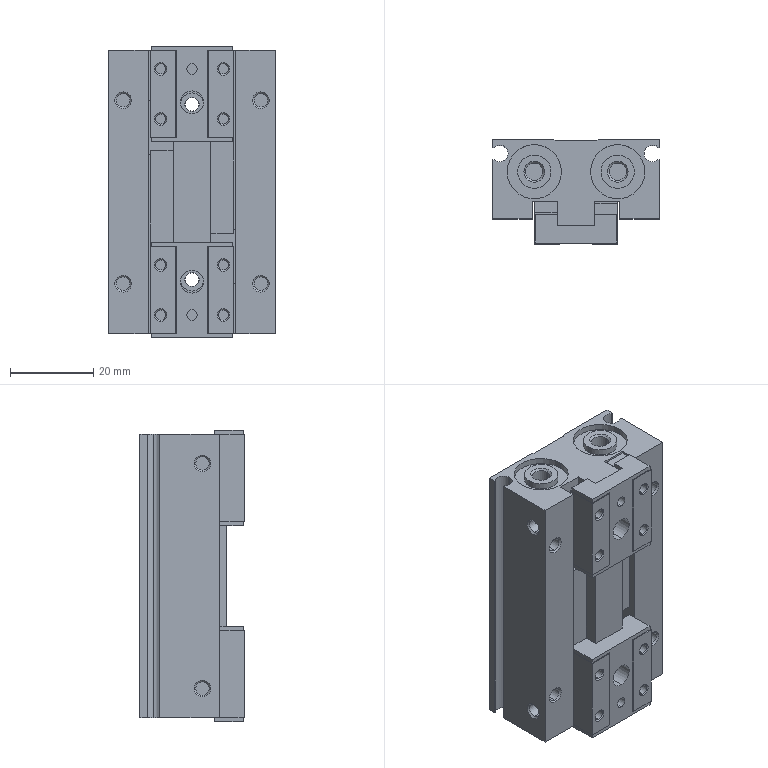Component | SolidWorks | MHF2-12D1_24_0-1 | 3 solids | 240 faces | box 40 x 25 x 70 mm | volume 51694 mm3 | plane 124 | cylinder 76 | cone 40 | commonest cylinder face diameters 3.242 x20 2.459 x16 5.5 x8 13 x8 3 x5 2.5 x4 8 x4 3.4 x4